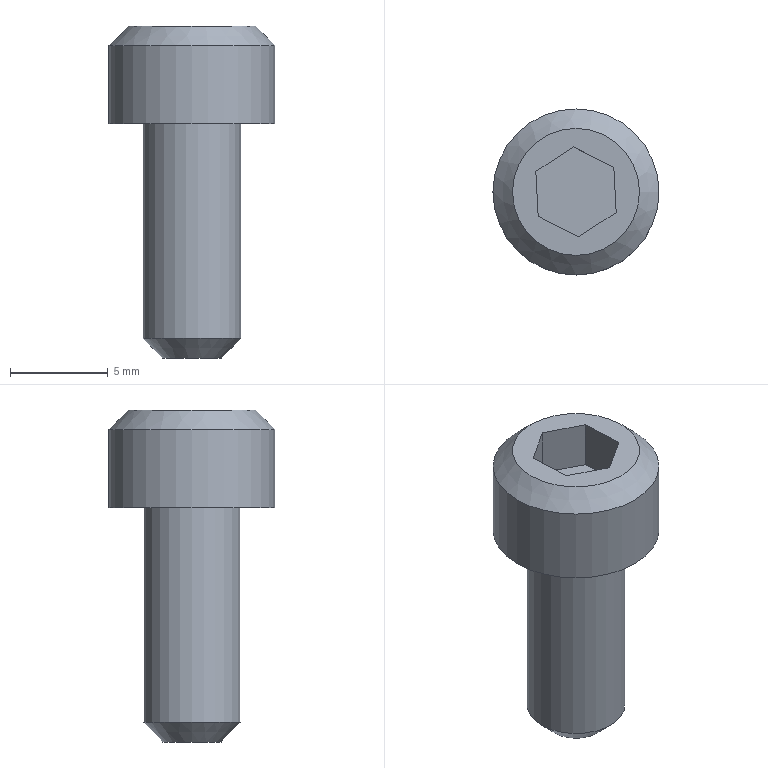Component | NX | HEX_SOCKET_SCREW_3 | 1 solid | 14 faces | box 8.5 x 8.5 x 17 mm | volume 466 mm3 | plane 10 | cylinder 2 | cone 2 | commonest cylinder face diameters 8.5 x1 5 x1
STEP:
#1=CARTESIAN_POINT('',(0.,0.,0.));
#2=DIRECTION('',(0.,0.,1.));
#3=DIRECTION('',(1.,0.,0.));
#4=AXIS2_PLACEMENT_3D('',#1,#2,#3);
#5=CARTESIAN_POINT('',(-126.076,-179.11,97.));
#6=VERTEX_POINT('',#5);
#7=CARTESIAN_POINT('',(-130.326,-179.11,97.));
#8=DIRECTION('',(0.,0.,-1.));
#9=DIRECTION('',(1.,0.,0.));
#10=AXIS2_PLACEMENT_3D('',#7,#8,#9);
#11=CIRCLE('',#10,4.25);
#12=CARTESIAN_POINT('',(-130.326,-179.11,93.));
#13=DIRECTION('',(0.,0.,1.));
#14=DIRECTION('',(-1.,0.,0.));
#15=AXIS2_PLACEMENT_3D('',#12,#13,#14);
#16=CYLINDRICAL_SURFACE('',#15,4.25);
#17=CARTESIAN_POINT('',(9.425,4.));
#18=DIRECTION('',(-1.,0.));
#19=VECTOR('',#18,1.);
#20=LINE('',#17,#19);
#21=(GEOMETRIC_REPRESENTATION_CONTEXT(2)PARAMETRIC_REPRESENTATION_CONTEXT()REPRESENTATION_CONTEXT('',''));
#22=DEFINITIONAL_REPRESENTATION('',(#20),#21);
#23=PCURVE('',#16,#22);
#24=CARTESIAN_POINT('',(-130.326,-179.11,97.));
#25=DIRECTION('',(0.,0.,-1.));
#26=DIRECTION('',(1.,0.,0.));
#27=AXIS2_PLACEMENT_3D('',#24,#25,#26);
#28=CONICAL_SURFACE('',#27,4.25,0.7854);
#29=CARTESIAN_POINT('',(0.,0.));
#30=DIRECTION('',(1.,0.));
#31=VECTOR('',#30,1.);
#32=LINE('',#29,#31);
#33=(GEOMETRIC_REPRESENTATION_CONTEXT(2)PARAMETRIC_REPRESENTATION_CONTEXT()REPRESENTATION_CONTEXT('',''));
#34=DEFINITIONAL_REPRESENTATION('',(#32),#33);
#35=PCURVE('',#28,#34);
#36=SURFACE_CURVE('',#11,(#23,#35),.PCURVE_S1.);
#37=EDGE_CURVE('',#6,#6,#36,.T.);
#38=ORIENTED_EDGE('',*,*,#37,.T.);
#39=CARTESIAN_POINT('',(-126.076,-179.11,93.));
#40=VERTEX_POINT('',#39);
#41=CARTESIAN_POINT('',(-126.076,-179.11,93.));
#42=CARTESIAN_POINT('',(-126.076,-179.11,97.));
#43=B_SPLINE_CURVE_WITH_KNOTS('',1,(#41,#42),.UNSPECIFIED.,.F.,.F.,(2,2),(0.,4.),.PIECEWISE_BEZIER_KNOTS.);
#44=CARTESIAN_POINT('',(3.142,0.));
#45=DIRECTION('',(0.,1.));
#46=VECTOR('',#45,1.);
#47=LINE('',#44,#46);
#48=(GEOMETRIC_REPRESENTATION_CONTEXT(2)PARAMETRIC_REPRESENTATION_CONTEXT()REPRESENTATION_CONTEXT('',''));
#49=DEFINITIONAL_REPRESENTATION('',(#47),#48);
#50=PCURVE('',#16,#49);
#51=CARTESIAN_POINT('',(9.425,0.));
#52=DIRECTION('',(0.,1.));
#53=VECTOR('',#52,1.);
#54=LINE('',#51,#53);
#55=(GEOMETRIC_REPRESENTATION_CONTEXT(2)PARAMETRIC_REPRESENTATION_CONTEXT()REPRESENTATION_CONTEXT('',''));
#56=DEFINITIONAL_REPRESENTATION('',(#54),#55);
#57=PCURVE('',#16,#56);
#58=SEAM_CURVE('',#43,(#50,#57),.PCURVE_S1.);
#59=EDGE_CURVE('',#40,#6,#58,.T.);
#60=ORIENTED_EDGE('',*,*,#59,.F.);
#61=CARTESIAN_POINT('',(-130.326,-179.11,93.));
#62=DIRECTION('',(0.,0.,-1.));
#63=DIRECTION('',(1.,0.,0.));
#64=AXIS2_PLACEMENT_3D('',#61,#62,#63);
#65=CIRCLE('',#64,4.25);
#66=CARTESIAN_POINT('',(9.425,0.));
#67=DIRECTION('',(-1.,0.));
#68=VECTOR('',#67,1.);
#69=LINE('',#66,#68);
#70=(GEOMETRIC_REPRESENTATION_CONTEXT(2)PARAMETRIC_REPRESENTATION_CONTEXT()REPRESENTATION_CONTEXT('',''));
#71=DEFINITIONAL_REPRESENTATION('',(#69),#70);
#72=PCURVE('',#16,#71);
#73=CARTESIAN_POINT('',(-130.326,-179.11,93.));
#74=DIRECTION('',(0.,0.,-1.));
#75=DIRECTION('',(1.,0.,0.));
#76=AXIS2_PLACEMENT_3D('',#73,#74,#75);
#77=PLANE('',#76);
#78=CARTESIAN_POINT('',(0.,0.));
#79=DIRECTION('',(1.,0.));
#80=AXIS2_PLACEMENT_2D('',#78,#79);
#81=CIRCLE('',#80,4.25);
#82=(GEOMETRIC_REPRESENTATION_CONTEXT(2)PARAMETRIC_REPRESENTATION_CONTEXT()REPRESENTATION_CONTEXT('',''));
#83=DEFINITIONAL_REPRESENTATION('',(#81),#82);
#84=PCURVE('',#77,#83);
#85=SURFACE_CURVE('',#65,(#72,#84),.PCURVE_S1.);
#86=EDGE_CURVE('',#40,#40,#85,.T.);
#87=ORIENTED_EDGE('',*,*,#86,.F.);
#88=ORIENTED_EDGE('',*,*,#59,.T.);
#89=EDGE_LOOP('',(#38,#60,#87,#88));
#90=FACE_BOUND('',#89,.T.);
#91=ADVANCED_FACE('',(#90),#16,.T.);
#92=CARTESIAN_POINT('',(-127.826,-179.11,93.));
#93=VERTEX_POINT('',#92);
#94=CARTESIAN_POINT('',(-130.326,-179.11,93.));
#95=DIRECTION('',(0.,0.,-1.));
#96=DIRECTION('',(1.,0.,0.));
#97=AXIS2_PLACEMENT_3D('',#94,#95,#96);
#98=CIRCLE('',#97,2.5);
#99=CARTESIAN_POINT('',(0.,0.));
#100=DIRECTION('',(1.,0.));
#101=AXIS2_PLACEMENT_2D('',#99,#100);
#102=CIRCLE('',#101,2.5);
#103=(GEOMETRIC_REPRESENTATION_CONTEXT(2)PARAMETRIC_REPRESENTATION_CONTEXT()REPRESENTATION_CONTEXT('',''));
#104=DEFINITIONAL_REPRESENTATION('',(#102),#103);
#105=PCURVE('',#77,#104);
#106=CARTESIAN_POINT('',(-130.326,-179.11,81.));
#107=DIRECTION('',(0.,0.,1.));
#108=DIRECTION('',(-1.,0.,0.));
#109=AXIS2_PLACEMENT_3D('',#106,#107,#108);
#110=CYLINDRICAL_SURFACE('',#109,2.5);
#111=CARTESIAN_POINT('',(9.425,12.));
#112=DIRECTION('',(-1.,0.));
#113=VECTOR('',#112,1.);
#114=LINE('',#111,#113);
#115=(GEOMETRIC_REPRESENTATION_CONTEXT(2)PARAMETRIC_REPRESENTATION_CONTEXT()REPRESENTATION_CONTEXT('',''));
#116=DEFINITIONAL_REPRESENTATION('',(#114),#115);
#117=PCURVE('',#110,#116);
#118=SURFACE_CURVE('',#98,(#105,#117),.PCURVE_S1.);
#119=EDGE_CURVE('',#93,#93,#118,.T.);
#120=ORIENTED_EDGE('',*,*,#119,.F.);
#121=EDGE_LOOP('',(#120));
#122=FACE_BOUND('',#121,.T.);
#123=ORIENTED_EDGE('',*,*,#86,.T.);
#124=EDGE_LOOP('',(#123));
#125=FACE_BOUND('',#124,.T.);
#126=ADVANCED_FACE('',(#122,#125),#77,.T.);
#127=CARTESIAN_POINT('',(-127.076,-179.11,98.));
#128=VERTEX_POINT('',#127);
#129=CARTESIAN_POINT('',(-130.326,-179.11,98.));
#130=DIRECTION('',(0.,0.,1.));
#131=DIRECTION('',(1.,0.,0.));
#132=AXIS2_PLACEMENT_3D('',#129,#130,#131);
#133=CIRCLE('',#132,3.25);
#134=CARTESIAN_POINT('',(-130.326,-179.11,98.));
#135=DIRECTION('',(0.,0.,-1.));
#136=DIRECTION('',(1.,0.,0.));
#137=AXIS2_PLACEMENT_3D('',#134,#135,#136);
#138=PLANE('',#137);
#139=CARTESIAN_POINT('',(3.25,0.));
#140=CARTESIAN_POINT('',(3.25,-5.629));
#141=CARTESIAN_POINT('',(-1.625,-2.815));
#142=CARTESIAN_POINT('',(-6.5,-0.));
#143=CARTESIAN_POINT('',(-1.625,2.815));
#144=CARTESIAN_POINT('',(3.25,5.629));
#145=CARTESIAN_POINT('',(3.25,0.));
#146=(BOUNDED_CURVE()B_SPLINE_CURVE(2,(#139,#140,#141,#142,#143,#144,#145),.UNSPECIFIED.,.T.,.F.)B_SPLINE_CURVE_WITH_KNOTS((1,2,2,2,2,1),(-2.094,0.,2.094,4.189,6.283,8.378),.UNSPECIFIED.)CURVE()GEOMETRIC_REPRESENTATION_ITEM()RATIONAL_B_SPLINE_CURVE((1.,0.5,1.,0.5,1.,0.5,1.))REPRESENTATION_ITEM(''));
#147=(GEOMETRIC_REPRESENTATION_CONTEXT(2)PARAMETRIC_REPRESENTATION_CONTEXT()REPRESENTATION_CONTEXT('',''));
#148=DEFINITIONAL_REPRESENTATION('',(#146),#147);
#149=PCURVE('',#138,#148);
#150=CARTESIAN_POINT('',(6.283,-1.));
#151=DIRECTION('',(-1.,0.));
#152=VECTOR('',#151,1.);
#153=LINE('',#150,#152);
#154=(GEOMETRIC_REPRESENTATION_CONTEXT(2)PARAMETRIC_REPRESENTATION_CONTEXT()REPRESENTATION_CONTEXT('',''));
#155=DEFINITIONAL_REPRESENTATION('',(#153),#154);
#156=PCURVE('',#28,#155);
#157=SURFACE_CURVE('',#133,(#149,#156),.PCURVE_S1.);
#158=EDGE_CURVE('',#128,#128,#157,.T.);
#159=ORIENTED_EDGE('',*,*,#158,.T.);
#160=EDGE_LOOP('',(#159));
#161=FACE_BOUND('',#160,.T.);
#162=CARTESIAN_POINT('',(-132.263,-180.368,98.));
#163=VERTEX_POINT('',#162);
#164=CARTESIAN_POINT('',(-130.205,-181.416,98.));
#165=VERTEX_POINT('',#164);
#166=CARTESIAN_POINT('',(-132.263,-180.368,98.));
#167=DIRECTION('',(0.891,-0.454,0.));
#168=VECTOR('',#167,1.);
#169=LINE('',#166,#168);
#170=CARTESIAN_POINT('',(-1.937,1.258));
#171=DIRECTION('',(0.891,0.454));
#172=VECTOR('',#171,1.);
#173=LINE('',#170,#172);
#174=(GEOMETRIC_REPRESENTATION_CONTEXT(2)PARAMETRIC_REPRESENTATION_CONTEXT()REPRESENTATION_CONTEXT('',''));
#175=DEFINITIONAL_REPRESENTATION('',(#173),#174);
#176=PCURVE('',#138,#175);
#177=CARTESIAN_POINT('',(-132.263,-180.368,95.5));
#178=DIRECTION('',(-0.454,-0.891,0.));
#179=DIRECTION('',(-0.891,0.454,0.));
#180=AXIS2_PLACEMENT_3D('',#177,#178,#179);
#181=PLANE('',#180);
#182=CARTESIAN_POINT('',(0.,-2.5));
#183=DIRECTION('',(-1.,0.));
#184=VECTOR('',#183,1.);
#185=LINE('',#182,#184);
#186=(GEOMETRIC_REPRESENTATION_CONTEXT(2)PARAMETRIC_REPRESENTATION_CONTEXT()REPRESENTATION_CONTEXT('',''));
#187=DEFINITIONAL_REPRESENTATION('',(#185),#186);
#188=PCURVE('',#181,#187);
#189=SURFACE_CURVE('',#169,(#176,#188),.PCURVE_S1.);
#190=EDGE_CURVE('',#163,#165,#189,.T.);
#191=ORIENTED_EDGE('',*,*,#190,.F.);
#192=CARTESIAN_POINT('',(-132.384,-178.062,98.));
#193=VERTEX_POINT('',#192);
#194=CARTESIAN_POINT('',(-132.384,-178.062,98.));
#195=DIRECTION('',(0.05234,-0.9986,0.));
#196=VECTOR('',#195,1.);
#197=LINE('',#194,#196);
#198=CARTESIAN_POINT('',(-2.058,-1.048));
#199=DIRECTION('',(0.05234,0.9986));
#200=VECTOR('',#199,1.);
#201=LINE('',#198,#200);
#202=(GEOMETRIC_REPRESENTATION_CONTEXT(2)PARAMETRIC_REPRESENTATION_CONTEXT()REPRESENTATION_CONTEXT('',''));
#203=DEFINITIONAL_REPRESENTATION('',(#201),#202);
#204=PCURVE('',#138,#203);
#205=CARTESIAN_POINT('',(-132.384,-178.062,95.5));
#206=DIRECTION('',(-0.9986,-0.05234,0.));
#207=DIRECTION('',(-0.05234,0.9986,0.));
#208=AXIS2_PLACEMENT_3D('',#205,#206,#207);
#209=PLANE('',#208);
#210=CARTESIAN_POINT('',(0.,-2.5));
#211=DIRECTION('',(-1.,0.));
#212=VECTOR('',#211,1.);
#213=LINE('',#210,#212);
#214=(GEOMETRIC_REPRESENTATION_CONTEXT(2)PARAMETRIC_REPRESENTATION_CONTEXT()REPRESENTATION_CONTEXT('',''));
#215=DEFINITIONAL_REPRESENTATION('',(#213),#214);
#216=PCURVE('',#209,#215);
#217=SURFACE_CURVE('',#197,(#204,#216),.PCURVE_S1.);
#218=EDGE_CURVE('',#193,#163,#217,.T.);
#219=ORIENTED_EDGE('',*,*,#218,.F.);
#220=CARTESIAN_POINT('',(-130.447,-176.804,98.));
#221=VERTEX_POINT('',#220);
#222=CARTESIAN_POINT('',(-130.447,-176.804,98.));
#223=DIRECTION('',(-0.8387,-0.5446,0.));
#224=VECTOR('',#223,1.);
#225=LINE('',#222,#224);
#226=CARTESIAN_POINT('',(-0.1209,-2.306));
#227=DIRECTION('',(-0.8387,0.5446));
#228=VECTOR('',#227,1.);
#229=LINE('',#226,#228);
#230=(GEOMETRIC_REPRESENTATION_CONTEXT(2)PARAMETRIC_REPRESENTATION_CONTEXT()REPRESENTATION_CONTEXT('',''));
#231=DEFINITIONAL_REPRESENTATION('',(#229),#230);
#232=PCURVE('',#138,#231);
#233=CARTESIAN_POINT('',(-130.447,-176.804,95.5));
#234=DIRECTION('',(-0.5446,0.8387,0.));
#235=DIRECTION('',(0.8387,0.5446,0.));
#236=AXIS2_PLACEMENT_3D('',#233,#234,#235);
#237=PLANE('',#236);
#238=CARTESIAN_POINT('',(0.,-2.5));
#239=DIRECTION('',(-1.,0.));
#240=VECTOR('',#239,1.);
#241=LINE('',#238,#240);
#242=(GEOMETRIC_REPRESENTATION_CONTEXT(2)PARAMETRIC_REPRESENTATION_CONTEXT()REPRESENTATION_CONTEXT('',''));
#243=DEFINITIONAL_REPRESENTATION('',(#241),#242);
#244=PCURVE('',#237,#243);
#245=SURFACE_CURVE('',#225,(#232,#244),.PCURVE_S1.);
#246=EDGE_CURVE('',#221,#193,#245,.T.);
#247=ORIENTED_EDGE('',*,*,#246,.F.);
#248=CARTESIAN_POINT('',(-128.389,-177.852,98.));
#249=VERTEX_POINT('',#248);
#250=CARTESIAN_POINT('',(-128.389,-177.852,98.));
#251=DIRECTION('',(-0.891,0.454,0.));
#252=VECTOR('',#251,1.);
#253=LINE('',#250,#252);
#254=CARTESIAN_POINT('',(1.937,-1.258));
#255=DIRECTION('',(-0.891,-0.454));
#256=VECTOR('',#255,1.);
#257=LINE('',#254,#256);
#258=(GEOMETRIC_REPRESENTATION_CONTEXT(2)PARAMETRIC_REPRESENTATION_CONTEXT()REPRESENTATION_CONTEXT('',''));
#259=DEFINITIONAL_REPRESENTATION('',(#257),#258);
#260=PCURVE('',#138,#259);
#261=CARTESIAN_POINT('',(-128.389,-177.852,95.5));
#262=DIRECTION('',(0.454,0.891,0.));
#263=DIRECTION('',(0.891,-0.454,0.));
#264=AXIS2_PLACEMENT_3D('',#261,#262,#263);
#265=PLANE('',#264);
#266=CARTESIAN_POINT('',(0.,-2.5));
#267=DIRECTION('',(-1.,0.));
#268=VECTOR('',#267,1.);
#269=LINE('',#266,#268);
#270=(GEOMETRIC_REPRESENTATION_CONTEXT(2)PARAMETRIC_REPRESENTATION_CONTEXT()REPRESENTATION_CONTEXT('',''));
#271=DEFINITIONAL_REPRESENTATION('',(#269),#270);
#272=PCURVE('',#265,#271);
#273=SURFACE_CURVE('',#253,(#260,#272),.PCURVE_S1.);
#274=EDGE_CURVE('',#249,#221,#273,.T.);
#275=ORIENTED_EDGE('',*,*,#274,.F.);
#276=CARTESIAN_POINT('',(-128.269,-180.158,98.));
#277=VERTEX_POINT('',#276);
#278=CARTESIAN_POINT('',(-128.269,-180.158,98.));
#279=DIRECTION('',(-0.05234,0.9986,0.));
#280=VECTOR('',#279,1.);
#281=LINE('',#278,#280);
#282=CARTESIAN_POINT('',(2.058,1.048));
#283=DIRECTION('',(-0.05234,-0.9986));
#284=VECTOR('',#283,1.);
#285=LINE('',#282,#284);
#286=(GEOMETRIC_REPRESENTATION_CONTEXT(2)PARAMETRIC_REPRESENTATION_CONTEXT()REPRESENTATION_CONTEXT('',''));
#287=DEFINITIONAL_REPRESENTATION('',(#285),#286);
#288=PCURVE('',#138,#287);
#289=CARTESIAN_POINT('',(-128.269,-180.158,95.5));
#290=DIRECTION('',(0.9986,0.05234,0.));
#291=DIRECTION('',(0.05234,-0.9986,0.));
#292=AXIS2_PLACEMENT_3D('',#289,#290,#291);
#293=PLANE('',#292);
#294=CARTESIAN_POINT('',(0.,-2.5));
#295=DIRECTION('',(-1.,0.));
#296=VECTOR('',#295,1.);
#297=LINE('',#294,#296);
#298=(GEOMETRIC_REPRESENTATION_CONTEXT(2)PARAMETRIC_REPRESENTATION_CONTEXT()REPRESENTATION_CONTEXT('',''));
#299=DEFINITIONAL_REPRESENTATION('',(#297),#298);
#300=PCURVE('',#293,#299);
#301=SURFACE_CURVE('',#281,(#288,#300),.PCURVE_S1.);
#302=EDGE_CURVE('',#277,#249,#301,.T.);
#303=ORIENTED_EDGE('',*,*,#302,.F.);
#304=CARTESIAN_POINT('',(-130.205,-181.416,98.));
#305=DIRECTION('',(0.8387,0.5446,0.));
#306=VECTOR('',#305,1.);
#307=LINE('',#304,#306);
#308=CARTESIAN_POINT('',(0.1209,2.306));
#309=DIRECTION('',(0.8387,-0.5446));
#310=VECTOR('',#309,1.);
#311=LINE('',#308,#310);
#312=(GEOMETRIC_REPRESENTATION_CONTEXT(2)PARAMETRIC_REPRESENTATION_CONTEXT()REPRESENTATION_CONTEXT('',''));
#313=DEFINITIONAL_REPRESENTATION('',(#311),#312);
#314=PCURVE('',#138,#313);
#315=CARTESIAN_POINT('',(-130.205,-181.416,95.5));
#316=DIRECTION('',(0.5446,-0.8387,0.));
#317=DIRECTION('',(-0.8387,-0.5446,0.));
#318=AXIS2_PLACEMENT_3D('',#315,#316,#317);
#319=PLANE('',#318);
#320=CARTESIAN_POINT('',(0.,-2.5));
#321=DIRECTION('',(-1.,0.));
#322=VECTOR('',#321,1.);
#323=LINE('',#320,#322);
#324=(GEOMETRIC_REPRESENTATION_CONTEXT(2)PARAMETRIC_REPRESENTATION_CONTEXT()REPRESENTATION_CONTEXT('',''));
#325=DEFINITIONAL_REPRESENTATION('',(#323),#324);
#326=PCURVE('',#319,#325);
#327=SURFACE_CURVE('',#307,(#314,#326),.PCURVE_S1.);
#328=EDGE_CURVE('',#165,#277,#327,.T.);
#329=ORIENTED_EDGE('',*,*,#328,.F.);
#330=EDGE_LOOP('',(#191,#219,#247,#275,#303,#329));
#331=FACE_BOUND('',#330,.T.);
#332=ADVANCED_FACE('',(#161,#331),#138,.F.);
#333=CARTESIAN_POINT('',(-127.826,-179.11,82.));
#334=VERTEX_POINT('',#333);
#335=CARTESIAN_POINT('',(-130.326,-179.11,82.));
#336=DIRECTION('',(0.,0.,1.));
#337=DIRECTION('',(1.,0.,0.));
#338=AXIS2_PLACEMENT_3D('',#335,#336,#337);
#339=CIRCLE('',#338,2.5);
#340=CARTESIAN_POINT('',(3.142,1.));
#341=DIRECTION('',(1.,0.));
#342=VECTOR('',#341,1.);
#343=LINE('',#340,#342);
#344=(GEOMETRIC_REPRESENTATION_CONTEXT(2)PARAMETRIC_REPRESENTATION_CONTEXT()REPRESENTATION_CONTEXT('',''));
#345=DEFINITIONAL_REPRESENTATION('',(#343),#344);
#346=PCURVE('',#110,#345);
#347=CARTESIAN_POINT('',(-130.326,-179.11,81.));
#348=DIRECTION('',(0.,0.,1.));
#349=DIRECTION('',(-1.,0.,0.));
#350=AXIS2_PLACEMENT_3D('',#347,#348,#349);
#351=CONICAL_SURFACE('',#350,1.5,0.7854);
#352=CARTESIAN_POINT('',(3.142,1.));
#353=DIRECTION('',(1.,0.));
#354=VECTOR('',#353,1.);
#355=LINE('',#352,#354);
#356=(GEOMETRIC_REPRESENTATION_CONTEXT(2)PARAMETRIC_REPRESENTATION_CONTEXT()REPRESENTATION_CONTEXT('',''));
#357=DEFINITIONAL_REPRESENTATION('',(#355),#356);
#358=PCURVE('',#351,#357);
#359=SURFACE_CURVE('',#339,(#346,#358),.PCURVE_S1.);
#360=EDGE_CURVE('',#334,#334,#359,.T.);
#361=ORIENTED_EDGE('',*,*,#360,.T.);
#362=CARTESIAN_POINT('',(-127.826,-179.11,82.));
#363=CARTESIAN_POINT('',(-127.826,-179.11,93.));
#364=B_SPLINE_CURVE_WITH_KNOTS('',1,(#362,#363),.UNSPECIFIED.,.F.,.F.,(2,2),(1.,12.),.PIECEWISE_BEZIER_KNOTS.);
#365=CARTESIAN_POINT('',(9.425,0.));
#366=DIRECTION('',(0.,1.));
#367=VECTOR('',#366,1.);
#368=LINE('',#365,#367);
#369=(GEOMETRIC_REPRESENTATION_CONTEXT(2)PARAMETRIC_REPRESENTATION_CONTEXT()REPRESENTATION_CONTEXT('',''));
#370=DEFINITIONAL_REPRESENTATION('',(#368),#369);
#371=PCURVE('',#110,#370);
#372=CARTESIAN_POINT('',(3.142,0.));
#373=DIRECTION('',(0.,1.));
#374=VECTOR('',#373,1.);
#375=LINE('',#372,#374);
#376=(GEOMETRIC_REPRESENTATION_CONTEXT(2)PARAMETRIC_REPRESENTATION_CONTEXT()REPRESENTATION_CONTEXT('',''));
#377=DEFINITIONAL_REPRESENTATION('',(#375),#376);
#378=PCURVE('',#110,#377);
#379=SEAM_CURVE('',#364,(#371,#378),.PCURVE_S1.);
#380=EDGE_CURVE('',#334,#93,#379,.T.);
#381=ORIENTED_EDGE('',*,*,#380,.T.);
#382=ORIENTED_EDGE('',*,*,#119,.T.);
#383=ORIENTED_EDGE('',*,*,#380,.F.);
#384=EDGE_LOOP('',(#361,#381,#382,#383));
#385=FACE_BOUND('',#384,.T.);
#386=ADVANCED_FACE('',(#385),#110,.T.);
#387=CARTESIAN_POINT('',(-128.826,-179.11,81.));
#388=VERTEX_POINT('',#387);
#389=CARTESIAN_POINT('',(-130.326,-179.11,81.));
#390=DIRECTION('',(0.,0.,-1.));
#391=DIRECTION('',(1.,0.,0.));
#392=AXIS2_PLACEMENT_3D('',#389,#390,#391);
#393=CIRCLE('',#392,1.5);
#394=CARTESIAN_POINT('',(-130.326,-179.11,81.));
#395=DIRECTION('',(0.,0.,-1.));
#396=DIRECTION('',(1.,0.,0.));
#397=AXIS2_PLACEMENT_3D('',#394,#395,#396);
#398=PLANE('',#397);
#399=CARTESIAN_POINT('',(0.,0.));
#400=DIRECTION('',(1.,0.));
#401=AXIS2_PLACEMENT_2D('',#399,#400);
#402=CIRCLE('',#401,1.5);
#403=(GEOMETRIC_REPRESENTATION_CONTEXT(2)PARAMETRIC_REPRESENTATION_CONTEXT()REPRESENTATION_CONTEXT('',''));
#404=DEFINITIONAL_REPRESENTATION('',(#402),#403);
#405=PCURVE('',#398,#404);
#406=CARTESIAN_POINT('',(9.425,0.));
#407=DIRECTION('',(-1.,0.));
#408=VECTOR('',#407,1.);
#409=LINE('',#406,#408);
#410=(GEOMETRIC_REPRESENTATION_CONTEXT(2)PARAMETRIC_REPRESENTATION_CONTEXT()REPRESENTATION_CONTEXT('',''));
#411=DEFINITIONAL_REPRESENTATION('',(#409),#410);
#412=PCURVE('',#351,#411);
#413=SURFACE_CURVE('',#393,(#405,#412),.PCURVE_S1.);
#414=EDGE_CURVE('',#388,#388,#413,.T.);
#415=ORIENTED_EDGE('',*,*,#414,.T.);
#416=EDGE_LOOP('',(#415));
#417=FACE_BOUND('',#416,.T.);
#418=ADVANCED_FACE('',(#417),#398,.T.);
#419=ORIENTED_EDGE('',*,*,#218,.T.);
#420=CARTESIAN_POINT('',(-132.263,-180.368,95.5));
#421=VERTEX_POINT('',#420);
#422=CARTESIAN_POINT('',(-132.263,-180.368,95.5));
#423=DIRECTION('',(0.,0.,1.));
#424=VECTOR('',#423,1.);
#425=LINE('',#422,#424);
#426=CARTESIAN_POINT('',(-2.309,0.));
#427=DIRECTION('',(0.,-1.));
#428=VECTOR('',#427,1.);
#429=LINE('',#426,#428);
#430=(GEOMETRIC_REPRESENTATION_CONTEXT(2)PARAMETRIC_REPRESENTATION_CONTEXT()REPRESENTATION_CONTEXT('',''));
#431=DEFINITIONAL_REPRESENTATION('',(#429),#430);
#432=PCURVE('',#209,#431);
#433=CARTESIAN_POINT('',(0.,0.));
#434=DIRECTION('',(0.,-1.));
#435=VECTOR('',#434,1.);
#436=LINE('',#433,#435);
#437=(GEOMETRIC_REPRESENTATION_CONTEXT(2)PARAMETRIC_REPRESENTATION_CONTEXT()REPRESENTATION_CONTEXT('',''));
#438=DEFINITIONAL_REPRESENTATION('',(#436),#437);
#439=PCURVE('',#181,#438);
#440=SURFACE_CURVE('',#425,(#432,#439),.PCURVE_S1.);
#441=EDGE_CURVE('',#421,#163,#440,.T.);
#442=ORIENTED_EDGE('',*,*,#441,.F.);
#443=CARTESIAN_POINT('',(-132.384,-178.062,95.5));
#444=VERTEX_POINT('',#443);
#445=CARTESIAN_POINT('',(-132.384,-178.062,95.5));
#446=DIRECTION('',(0.05234,-0.9986,0.));
#447=VECTOR('',#446,1.);
#448=LINE('',#445,#447);
#449=CARTESIAN_POINT('',(0.,0.));
#450=DIRECTION('',(-1.,0.));
#451=VECTOR('',#450,1.);
#452=LINE('',#449,#451);
#453=(GEOMETRIC_REPRESENTATION_CONTEXT(2)PARAMETRIC_REPRESENTATION_CONTEXT()REPRESENTATION_CONTEXT('',''));
#454=DEFINITIONAL_REPRESENTATION('',(#452),#453);
#455=PCURVE('',#209,#454);
#456=CARTESIAN_POINT('',(-130.326,-179.11,95.5));
#457=DIRECTION('',(0.,0.,1.));
#458=DIRECTION('',(-1.,0.,0.));
#459=AXIS2_PLACEMENT_3D('',#456,#457,#458);
#460=PLANE('',#459);
#461=CARTESIAN_POINT('',(2.058,-1.048));
#462=DIRECTION('',(-0.05234,0.9986));
#463=VECTOR('',#462,1.);
#464=LINE('',#461,#463);
#465=(GEOMETRIC_REPRESENTATION_CONTEXT(2)PARAMETRIC_REPRESENTATION_CONTEXT()REPRESENTATION_CONTEXT('',''));
#466=DEFINITIONAL_REPRESENTATION('',(#464),#465);
#467=PCURVE('',#460,#466);
#468=SURFACE_CURVE('',#448,(#455,#467),.PCURVE_S1.);
#469=EDGE_CURVE('',#444,#421,#468,.T.);
#470=ORIENTED_EDGE('',*,*,#469,.F.);
#471=CARTESIAN_POINT('',(-132.384,-178.062,95.5));
#472=DIRECTION('',(0.,0.,1.));
#473=VECTOR('',#472,1.);
#474=LINE('',#471,#473);
#475=CARTESIAN_POINT('',(0.,0.));
#476=DIRECTION('',(0.,-1.));
#477=VECTOR('',#476,1.);
#478=LINE('',#475,#477);
#479=(GEOMETRIC_REPRESENTATION_CONTEXT(2)PARAMETRIC_REPRESENTATION_CONTEXT()REPRESENTATION_CONTEXT('',''));
#480=DEFINITIONAL_REPRESENTATION('',(#478),#479);
#481=PCURVE('',#209,#480);
#482=CARTESIAN_POINT('',(-2.309,0.));
#483=DIRECTION('',(0.,-1.));
#484=VECTOR('',#483,1.);
#485=LINE('',#482,#484);
#486=(GEOMETRIC_REPRESENTATION_CONTEXT(2)PARAMETRIC_REPRESENTATION_CONTEXT()REPRESENTATION_CONTEXT('',''));
#487=DEFINITIONAL_REPRESENTATION('',(#485),#486);
#488=PCURVE('',#237,#487);
#489=SURFACE_CURVE('',#474,(#481,#488),.PCURVE_S1.);
#490=EDGE_CURVE('',#444,#193,#489,.T.);
#491=ORIENTED_EDGE('',*,*,#490,.T.);
#492=EDGE_LOOP('',(#419,#442,#470,#491));
#493=FACE_BOUND('',#492,.T.);
#494=ADVANCED_FACE('',(#493),#209,.F.);
#495=ORIENTED_EDGE('',*,*,#190,.T.);
#496=CARTESIAN_POINT('',(-130.205,-181.416,95.5));
#497=VERTEX_POINT('',#496);
#498=CARTESIAN_POINT('',(-130.205,-181.416,95.5));
#499=DIRECTION('',(0.,0.,1.));
#500=VECTOR('',#499,1.);
#501=LINE('',#498,#500);
#502=CARTESIAN_POINT('',(-2.309,0.));
#503=DIRECTION('',(0.,-1.));
#504=VECTOR('',#503,1.);
#505=LINE('',#502,#504);
#506=(GEOMETRIC_REPRESENTATION_CONTEXT(2)PARAMETRIC_REPRESENTATION_CONTEXT()REPRESENTATION_CONTEXT('',''));
#507=DEFINITIONAL_REPRESENTATION('',(#505),#506);
#508=PCURVE('',#181,#507);
#509=CARTESIAN_POINT('',(0.,0.));
#510=DIRECTION('',(0.,-1.));
#511=VECTOR('',#510,1.);
#512=LINE('',#509,#511);
#513=(GEOMETRIC_REPRESENTATION_CONTEXT(2)PARAMETRIC_REPRESENTATION_CONTEXT()REPRESENTATION_CONTEXT('',''));
#514=DEFINITIONAL_REPRESENTATION('',(#512),#513);
#515=PCURVE('',#319,#514);
#516=SURFACE_CURVE('',#501,(#508,#515),.PCURVE_S1.);
#517=EDGE_CURVE('',#497,#165,#516,.T.);
#518=ORIENTED_EDGE('',*,*,#517,.F.);
#519=CARTESIAN_POINT('',(-132.263,-180.368,95.5));
#520=DIRECTION('',(0.891,-0.454,0.));
#521=VECTOR('',#520,1.);
#522=LINE('',#519,#521);
#523=CARTESIAN_POINT('',(0.,0.));
#524=DIRECTION('',(-1.,0.));
#525=VECTOR('',#524,1.);
#526=LINE('',#523,#525);
#527=(GEOMETRIC_REPRESENTATION_CONTEXT(2)PARAMETRIC_REPRESENTATION_CONTEXT()REPRESENTATION_CONTEXT('',''));
#528=DEFINITIONAL_REPRESENTATION('',(#526),#527);
#529=PCURVE('',#181,#528);
#530=CARTESIAN_POINT('',(1.937,1.258));
#531=DIRECTION('',(-0.891,0.454));
#532=VECTOR('',#531,1.);
#533=LINE('',#530,#532);
#534=(GEOMETRIC_REPRESENTATION_CONTEXT(2)PARAMETRIC_REPRESENTATION_CONTEXT()REPRESENTATION_CONTEXT('',''));
#535=DEFINITIONAL_REPRESENTATION('',(#533),#534);
#536=PCURVE('',#460,#535);
#537=SURFACE_CURVE('',#522,(#529,#536),.PCURVE_S1.);
#538=EDGE_CURVE('',#421,#497,#537,.T.);
#539=ORIENTED_EDGE('',*,*,#538,.F.);
#540=ORIENTED_EDGE('',*,*,#441,.T.);
#541=EDGE_LOOP('',(#495,#518,#539,#540));
#542=FACE_BOUND('',#541,.T.);
#543=ADVANCED_FACE('',(#542),#181,.F.);
#544=ORIENTED_EDGE('',*,*,#328,.T.);
#545=CARTESIAN_POINT('',(-128.269,-180.158,95.5));
#546=VERTEX_POINT('',#545);
#547=CARTESIAN_POINT('',(-128.269,-180.158,95.5));
#548=DIRECTION('',(0.,0.,1.));
#549=VECTOR('',#548,1.);
#550=LINE('',#547,#549);
#551=CARTESIAN_POINT('',(-2.309,0.));
#552=DIRECTION('',(0.,-1.));
#553=VECTOR('',#552,1.);
#554=LINE('',#551,#553);
#555=(GEOMETRIC_REPRESENTATION_CONTEXT(2)PARAMETRIC_REPRESENTATION_CONTEXT()REPRESENTATION_CONTEXT('',''));
#556=DEFINITIONAL_REPRESENTATION('',(#554),#555);
#557=PCURVE('',#319,#556);
#558=CARTESIAN_POINT('',(0.,0.));
#559=DIRECTION('',(0.,-1.));
#560=VECTOR('',#559,1.);
#561=LINE('',#558,#560);
#562=(GEOMETRIC_REPRESENTATION_CONTEXT(2)PARAMETRIC_REPRESENTATION_CONTEXT()REPRESENTATION_CONTEXT('',''));
#563=DEFINITIONAL_REPRESENTATION('',(#561),#562);
#564=PCURVE('',#293,#563);
#565=SURFACE_CURVE('',#550,(#557,#564),.PCURVE_S1.);
#566=EDGE_CURVE('',#546,#277,#565,.T.);
#567=ORIENTED_EDGE('',*,*,#566,.F.);
#568=CARTESIAN_POINT('',(-130.205,-181.416,95.5));
#569=DIRECTION('',(0.8387,0.5446,0.));
#570=VECTOR('',#569,1.);
#571=LINE('',#568,#570);
#572=CARTESIAN_POINT('',(0.,0.));
#573=DIRECTION('',(-1.,0.));
#574=VECTOR('',#573,1.);
#575=LINE('',#572,#574);
#576=(GEOMETRIC_REPRESENTATION_CONTEXT(2)PARAMETRIC_REPRESENTATION_CONTEXT()REPRESENTATION_CONTEXT('',''));
#577=DEFINITIONAL_REPRESENTATION('',(#575),#576);
#578=PCURVE('',#319,#577);
#579=CARTESIAN_POINT('',(-0.1209,2.306));
#580=DIRECTION('',(-0.8387,-0.5446));
#581=VECTOR('',#580,1.);
#582=LINE('',#579,#581);
#583=(GEOMETRIC_REPRESENTATION_CONTEXT(2)PARAMETRIC_REPRESENTATION_CONTEXT()REPRESENTATION_CONTEXT('',''));
#584=DEFINITIONAL_REPRESENTATION('',(#582),#583);
#585=PCURVE('',#460,#584);
#586=SURFACE_CURVE('',#571,(#578,#585),.PCURVE_S1.);
#587=EDGE_CURVE('',#497,#546,#586,.T.);
#588=ORIENTED_EDGE('',*,*,#587,.F.);
#589=ORIENTED_EDGE('',*,*,#517,.T.);
#590=EDGE_LOOP('',(#544,#567,#588,#589));
#591=FACE_BOUND('',#590,.T.);
#592=ADVANCED_FACE('',(#591),#319,.F.);
#593=ORIENTED_EDGE('',*,*,#302,.T.);
#594=CARTESIAN_POINT('',(-128.389,-177.852,95.5));
#595=VERTEX_POINT('',#594);
#596=CARTESIAN_POINT('',(-128.389,-177.852,95.5));
#597=DIRECTION('',(0.,0.,1.));
#598=VECTOR('',#597,1.);
#599=LINE('',#596,#598);
#600=CARTESIAN_POINT('',(-2.309,0.));
#601=DIRECTION('',(0.,-1.));
#602=VECTOR('',#601,1.);
#603=LINE('',#600,#602);
#604=(GEOMETRIC_REPRESENTATION_CONTEXT(2)PARAMETRIC_REPRESENTATION_CONTEXT()REPRESENTATION_CONTEXT('',''));
#605=DEFINITIONAL_REPRESENTATION('',(#603),#604);
#606=PCURVE('',#293,#605);
#607=CARTESIAN_POINT('',(0.,0.));
#608=DIRECTION('',(0.,-1.));
#609=VECTOR('',#608,1.);
#610=LINE('',#607,#609);
#611=(GEOMETRIC_REPRESENTATION_CONTEXT(2)PARAMETRIC_REPRESENTATION_CONTEXT()REPRESENTATION_CONTEXT('',''));
#612=DEFINITIONAL_REPRESENTATION('',(#610),#611);
#613=PCURVE('',#265,#612);
#614=SURFACE_CURVE('',#599,(#606,#613),.PCURVE_S1.);
#615=EDGE_CURVE('',#595,#249,#614,.T.);
#616=ORIENTED_EDGE('',*,*,#615,.F.);
#617=CARTESIAN_POINT('',(-128.269,-180.158,95.5));
#618=DIRECTION('',(-0.05234,0.9986,0.));
#619=VECTOR('',#618,1.);
#620=LINE('',#617,#619);
#621=CARTESIAN_POINT('',(0.,0.));
#622=DIRECTION('',(-1.,0.));
#623=VECTOR('',#622,1.);
#624=LINE('',#621,#623);
#625=(GEOMETRIC_REPRESENTATION_CONTEXT(2)PARAMETRIC_REPRESENTATION_CONTEXT()REPRESENTATION_CONTEXT('',''));
#626=DEFINITIONAL_REPRESENTATION('',(#624),#625);
#627=PCURVE('',#293,#626);
#628=CARTESIAN_POINT('',(-2.058,1.048));
#629=DIRECTION('',(0.05234,-0.9986));
#630=VECTOR('',#629,1.);
#631=LINE('',#628,#630);
#632=(GEOMETRIC_REPRESENTATION_CONTEXT(2)PARAMETRIC_REPRESENTATION_CONTEXT()REPRESENTATION_CONTEXT('',''));
#633=DEFINITIONAL_REPRESENTATION('',(#631),#632);
#634=PCURVE('',#460,#633);
#635=SURFACE_CURVE('',#620,(#627,#634),.PCURVE_S1.);
#636=EDGE_CURVE('',#546,#595,#635,.T.);
#637=ORIENTED_EDGE('',*,*,#636,.F.);
#638=ORIENTED_EDGE('',*,*,#566,.T.);
#639=EDGE_LOOP('',(#593,#616,#637,#638));
#640=FACE_BOUND('',#639,.T.);
#641=ADVANCED_FACE('',(#640),#293,.F.);
#642=ORIENTED_EDGE('',*,*,#274,.T.);
#643=CARTESIAN_POINT('',(-130.447,-176.804,95.5));
#644=VERTEX_POINT('',#643);
#645=CARTESIAN_POINT('',(-130.447,-176.804,95.5));
#646=DIRECTION('',(0.,0.,1.));
#647=VECTOR('',#646,1.);
#648=LINE('',#645,#647);
#649=CARTESIAN_POINT('',(-2.309,0.));
#650=DIRECTION('',(0.,-1.));
#651=VECTOR('',#650,1.);
#652=LINE('',#649,#651);
#653=(GEOMETRIC_REPRESENTATION_CONTEXT(2)PARAMETRIC_REPRESENTATION_CONTEXT()REPRESENTATION_CONTEXT('',''));
#654=DEFINITIONAL_REPRESENTATION('',(#652),#653);
#655=PCURVE('',#265,#654);
#656=CARTESIAN_POINT('',(0.,0.));
#657=DIRECTION('',(0.,-1.));
#658=VECTOR('',#657,1.);
#659=LINE('',#656,#658);
#660=(GEOMETRIC_REPRESENTATION_CONTEXT(2)PARAMETRIC_REPRESENTATION_CONTEXT()REPRESENTATION_CONTEXT('',''));
#661=DEFINITIONAL_REPRESENTATION('',(#659),#660);
#662=PCURVE('',#237,#661);
#663=SURFACE_CURVE('',#648,(#655,#662),.PCURVE_S1.);
#664=EDGE_CURVE('',#644,#221,#663,.T.);
#665=ORIENTED_EDGE('',*,*,#664,.F.);
#666=CARTESIAN_POINT('',(-128.389,-177.852,95.5));
#667=DIRECTION('',(-0.891,0.454,0.));
#668=VECTOR('',#667,1.);
#669=LINE('',#666,#668);
#670=CARTESIAN_POINT('',(0.,0.));
#671=DIRECTION('',(-1.,0.));
#672=VECTOR('',#671,1.);
#673=LINE('',#670,#672);
#674=(GEOMETRIC_REPRESENTATION_CONTEXT(2)PARAMETRIC_REPRESENTATION_CONTEXT()REPRESENTATION_CONTEXT('',''));
#675=DEFINITIONAL_REPRESENTATION('',(#673),#674);
#676=PCURVE('',#265,#675);
#677=CARTESIAN_POINT('',(-1.937,-1.258));
#678=DIRECTION('',(0.891,-0.454));
#679=VECTOR('',#678,1.);
#680=LINE('',#677,#679);
#681=(GEOMETRIC_REPRESENTATION_CONTEXT(2)PARAMETRIC_REPRESENTATION_CONTEXT()REPRESENTATION_CONTEXT('',''));
#682=DEFINITIONAL_REPRESENTATION('',(#680),#681);
#683=PCURVE('',#460,#682);
#684=SURFACE_CURVE('',#669,(#676,#683),.PCURVE_S1.);
#685=EDGE_CURVE('',#595,#644,#684,.T.);
#686=ORIENTED_EDGE('',*,*,#685,.F.);
#687=ORIENTED_EDGE('',*,*,#615,.T.);
#688=EDGE_LOOP('',(#642,#665,#686,#687));
#689=FACE_BOUND('',#688,.T.);
#690=ADVANCED_FACE('',(#689),#265,.F.);
#691=ORIENTED_EDGE('',*,*,#246,.T.);
#692=ORIENTED_EDGE('',*,*,#490,.F.);
#693=CARTESIAN_POINT('',(-130.447,-176.804,95.5));
#694=DIRECTION('',(-0.8387,-0.5446,0.));
#695=VECTOR('',#694,1.);
#696=LINE('',#693,#695);
#697=CARTESIAN_POINT('',(0.,0.));
#698=DIRECTION('',(-1.,0.));
#699=VECTOR('',#698,1.);
#700=LINE('',#697,#699);
#701=(GEOMETRIC_REPRESENTATION_CONTEXT(2)PARAMETRIC_REPRESENTATION_CONTEXT()REPRESENTATION_CONTEXT('',''));
#702=DEFINITIONAL_REPRESENTATION('',(#700),#701);
#703=PCURVE('',#237,#702);
#704=CARTESIAN_POINT('',(0.1209,-2.306));
#705=DIRECTION('',(0.8387,0.5446));
#706=VECTOR('',#705,1.);
#707=LINE('',#704,#706);
#708=(GEOMETRIC_REPRESENTATION_CONTEXT(2)PARAMETRIC_REPRESENTATION_CONTEXT()REPRESENTATION_CONTEXT('',''));
#709=DEFINITIONAL_REPRESENTATION('',(#707),#708);
#710=PCURVE('',#460,#709);
#711=SURFACE_CURVE('',#696,(#703,#710),.PCURVE_S1.);
#712=EDGE_CURVE('',#644,#444,#711,.T.);
#713=ORIENTED_EDGE('',*,*,#712,.F.);
#714=ORIENTED_EDGE('',*,*,#664,.T.);
#715=EDGE_LOOP('',(#691,#692,#713,#714));
#716=FACE_BOUND('',#715,.T.);
#717=ADVANCED_FACE('',(#716),#237,.F.);
#718=ORIENTED_EDGE('',*,*,#469,.T.);
#719=ORIENTED_EDGE('',*,*,#538,.T.);
#720=ORIENTED_EDGE('',*,*,#587,.T.);
#721=ORIENTED_EDGE('',*,*,#636,.T.);
#722=ORIENTED_EDGE('',*,*,#685,.T.);
#723=ORIENTED_EDGE('',*,*,#712,.T.);
#724=EDGE_LOOP('',(#718,#719,#720,#721,#722,#723));
#725=FACE_BOUND('',#724,.T.);
#726=ADVANCED_FACE('',(#725),#460,.T.);
#727=ORIENTED_EDGE('',*,*,#360,.F.);
#728=CARTESIAN_POINT('',(-128.826,-179.11,81.));
#729=CARTESIAN_POINT('',(-127.826,-179.11,82.));
#730=B_SPLINE_CURVE_WITH_KNOTS('',1,(#728,#729),.UNSPECIFIED.,.F.,.F.,(2,2),(0.,1.414),.PIECEWISE_BEZIER_KNOTS.);
#731=CARTESIAN_POINT('',(3.142,0.));
#732=DIRECTION('',(0.,1.));
#733=VECTOR('',#732,1.);
#734=LINE('',#731,#733);
#735=(GEOMETRIC_REPRESENTATION_CONTEXT(2)PARAMETRIC_REPRESENTATION_CONTEXT()REPRESENTATION_CONTEXT('',''));
#736=DEFINITIONAL_REPRESENTATION('',(#734),#735);
#737=PCURVE('',#351,#736);
#738=CARTESIAN_POINT('',(9.425,0.));
#739=DIRECTION('',(0.,1.));
#740=VECTOR('',#739,1.);
#741=LINE('',#738,#740);
#742=(GEOMETRIC_REPRESENTATION_CONTEXT(2)PARAMETRIC_REPRESENTATION_CONTEXT()REPRESENTATION_CONTEXT('',''));
#743=DEFINITIONAL_REPRESENTATION('',(#741),#742);
#744=PCURVE('',#351,#743);
#745=SEAM_CURVE('',#730,(#737,#744),.PCURVE_S1.);
#746=EDGE_CURVE('',#388,#334,#745,.T.);
#747=ORIENTED_EDGE('',*,*,#746,.F.);
#748=ORIENTED_EDGE('',*,*,#414,.F.);
#749=ORIENTED_EDGE('',*,*,#746,.T.);
#750=EDGE_LOOP('',(#727,#747,#748,#749));
#751=FACE_BOUND('',#750,.T.);
#752=ADVANCED_FACE('',(#751),#351,.T.);
#753=ORIENTED_EDGE('',*,*,#158,.F.);
#754=CARTESIAN_POINT('',(-127.076,-179.11,98.));
#755=CARTESIAN_POINT('',(-126.076,-179.11,97.));
#756=B_SPLINE_CURVE_WITH_KNOTS('',1,(#754,#755),.UNSPECIFIED.,.F.,.F.,(2,2),(-1.414,0.),.PIECEWISE_BEZIER_KNOTS.);
#757=CARTESIAN_POINT('',(6.283,0.));
#758=DIRECTION('',(0.,1.));
#759=VECTOR('',#758,1.);
#760=LINE('',#757,#759);
#761=(GEOMETRIC_REPRESENTATION_CONTEXT(2)PARAMETRIC_REPRESENTATION_CONTEXT()REPRESENTATION_CONTEXT('',''));
#762=DEFINITIONAL_REPRESENTATION('',(#760),#761);
#763=PCURVE('',#28,#762);
#764=CARTESIAN_POINT('',(0.,0.));
#765=DIRECTION('',(0.,1.));
#766=VECTOR('',#765,1.);
#767=LINE('',#764,#766);
#768=(GEOMETRIC_REPRESENTATION_CONTEXT(2)PARAMETRIC_REPRESENTATION_CONTEXT()REPRESENTATION_CONTEXT('',''));
#769=DEFINITIONAL_REPRESENTATION('',(#767),#768);
#770=PCURVE('',#28,#769);
#771=SEAM_CURVE('',#756,(#763,#770),.PCURVE_S1.);
#772=EDGE_CURVE('',#128,#6,#771,.T.);
#773=ORIENTED_EDGE('',*,*,#772,.T.);
#774=ORIENTED_EDGE('',*,*,#37,.F.);
#775=ORIENTED_EDGE('',*,*,#772,.F.);
#776=EDGE_LOOP('',(#753,#773,#774,#775));
#777=FACE_BOUND('',#776,.T.);
#778=ADVANCED_FACE('',(#777),#28,.T.);
#779=CLOSED_SHELL('',(#91,#126,#332,#386,#418,#494,#543,#592,#641,#690,#717,#726,#752,#778));
#780=MANIFOLD_SOLID_BREP('',#779);
#781=(LENGTH_UNIT()NAMED_UNIT(*)SI_UNIT(.MILLI.,.METRE.));
#782=UNCERTAINTY_MEASURE_WITH_UNIT(LENGTH_MEASURE(0.000002),#781,'','');
#783=(NAMED_UNIT(*)PLANE_ANGLE_UNIT()SI_UNIT($,.RADIAN.));
#784=(NAMED_UNIT(*)SI_UNIT($,.STERADIAN.)SOLID_ANGLE_UNIT());
#785=(GEOMETRIC_REPRESENTATION_CONTEXT(3)GLOBAL_UNCERTAINTY_ASSIGNED_CONTEXT((#782))GLOBAL_UNIT_ASSIGNED_CONTEXT((#781,#783,#784))REPRESENTATION_CONTEXT('',''));
#786=ADVANCED_BREP_SHAPE_REPRESENTATION('',(#4,#780),#785);